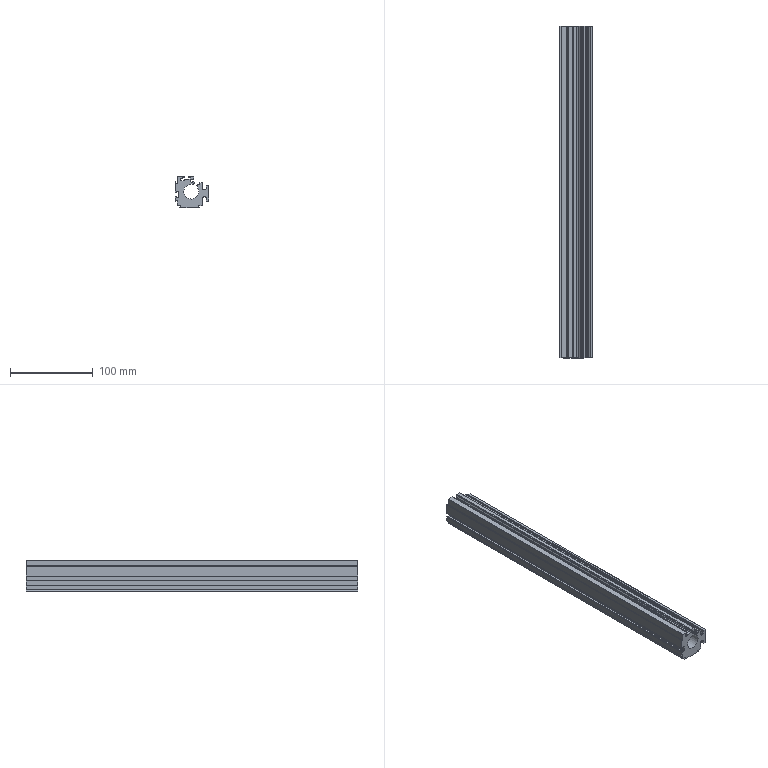Component | SolidWorks | DGC-18-280-G-PPV-A-1_532446 DGC-182804---00041181--(ZR)-1 | 1 solid | 112 faces | volume 347220 mm3 | cylinder 59 | plane 53 | commonest cylinder face diameters 0.6 x20 0.4 x11 1 x6 0.8 x5 3.2 x4 3 x4 0.66 x2 4.3 x2